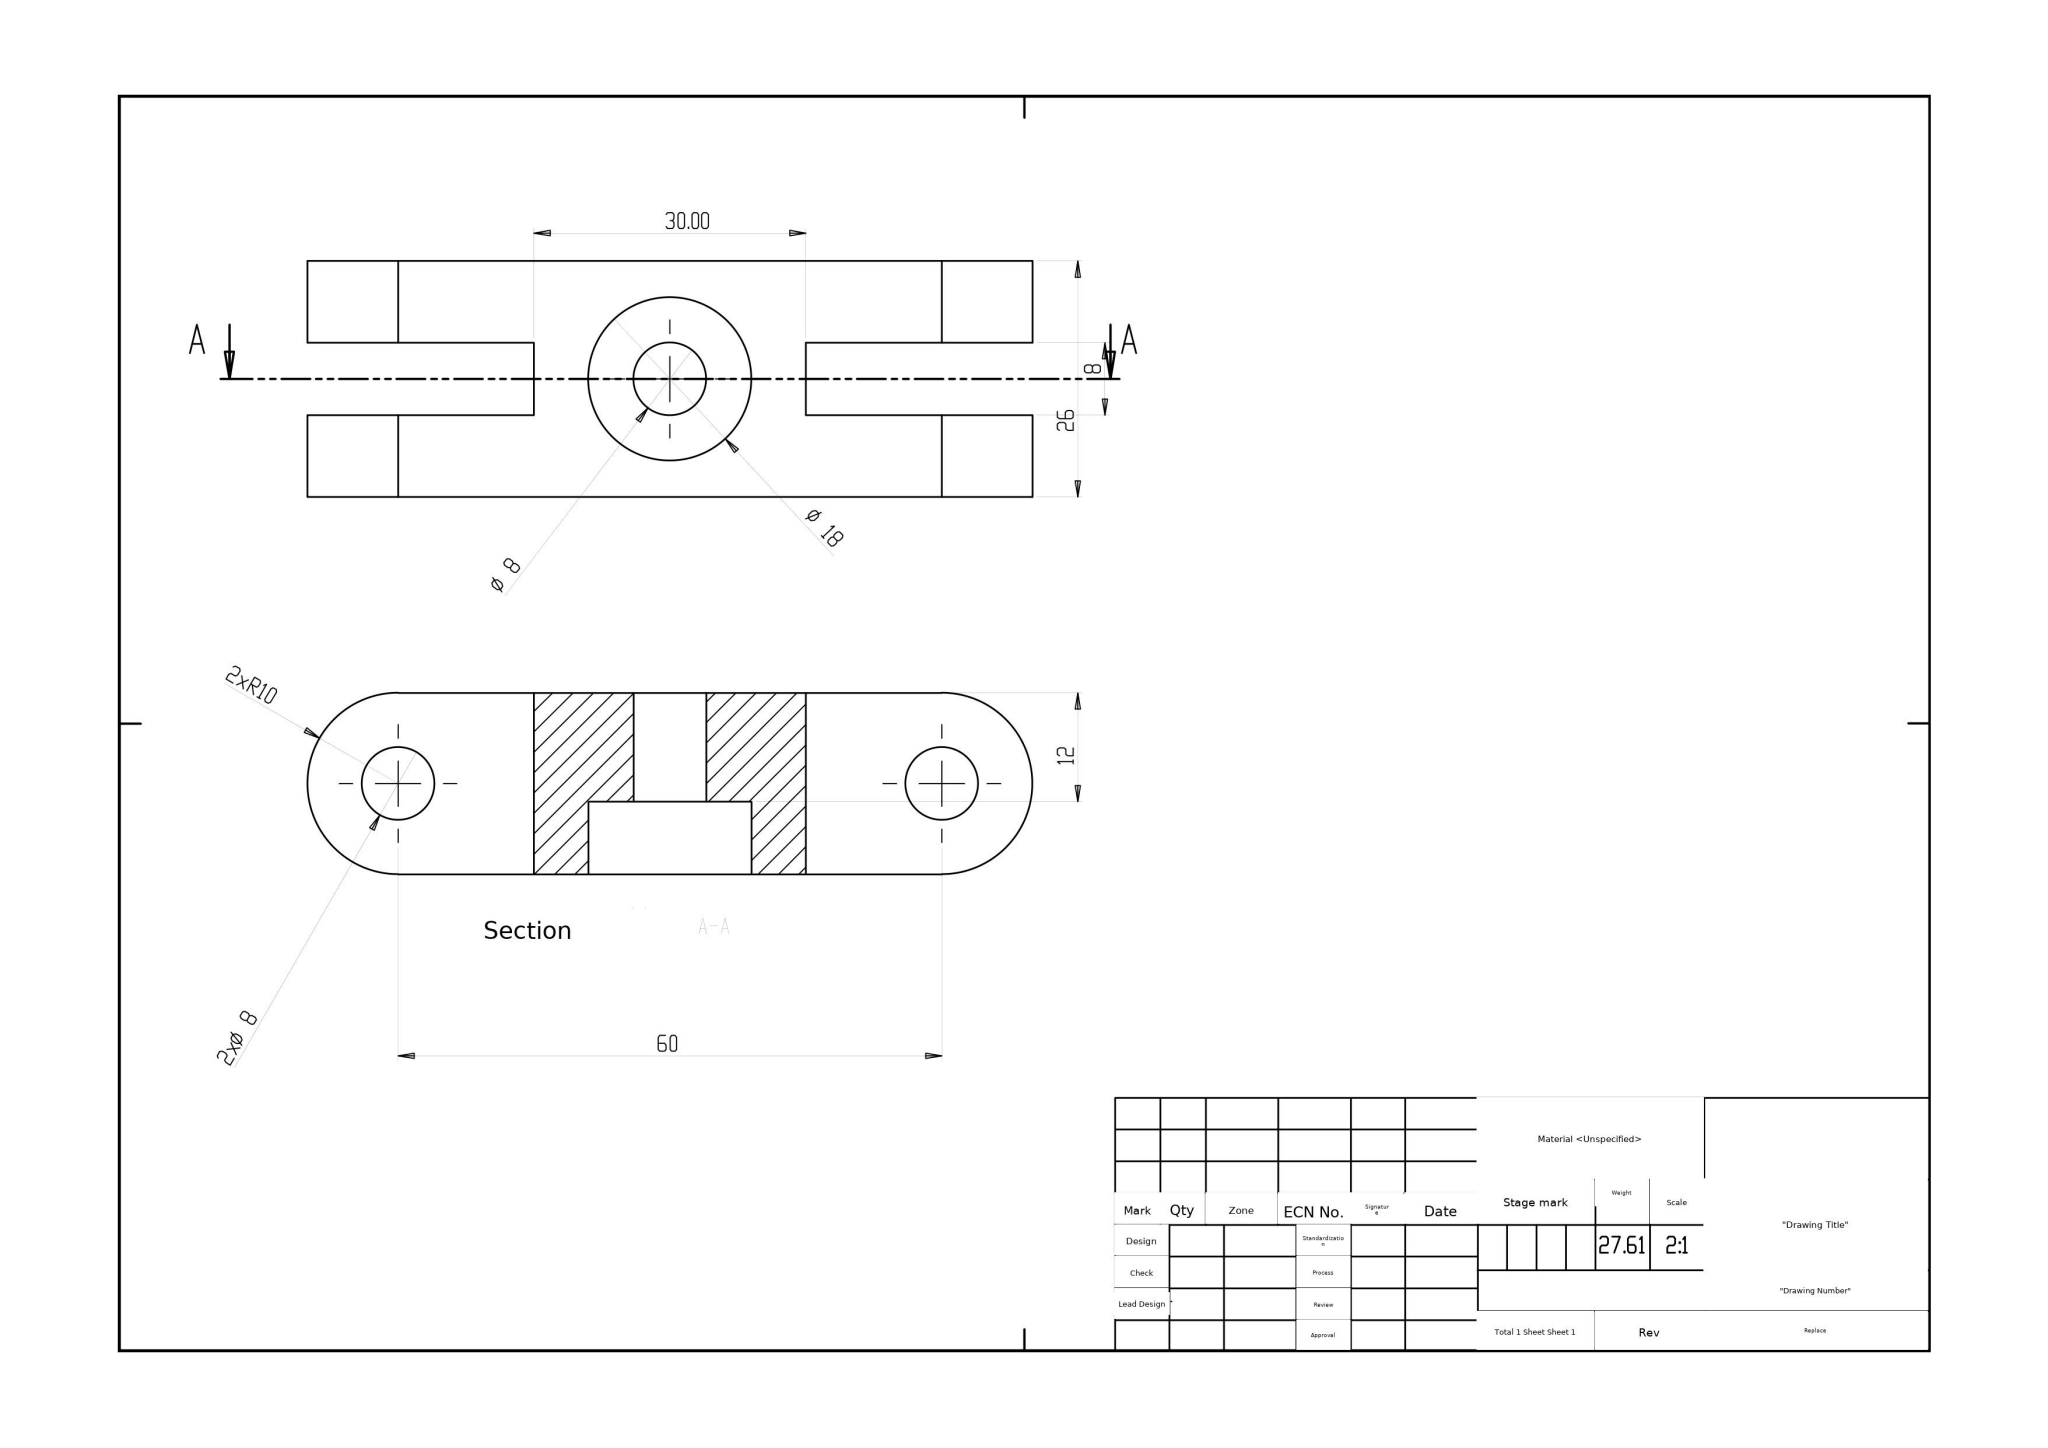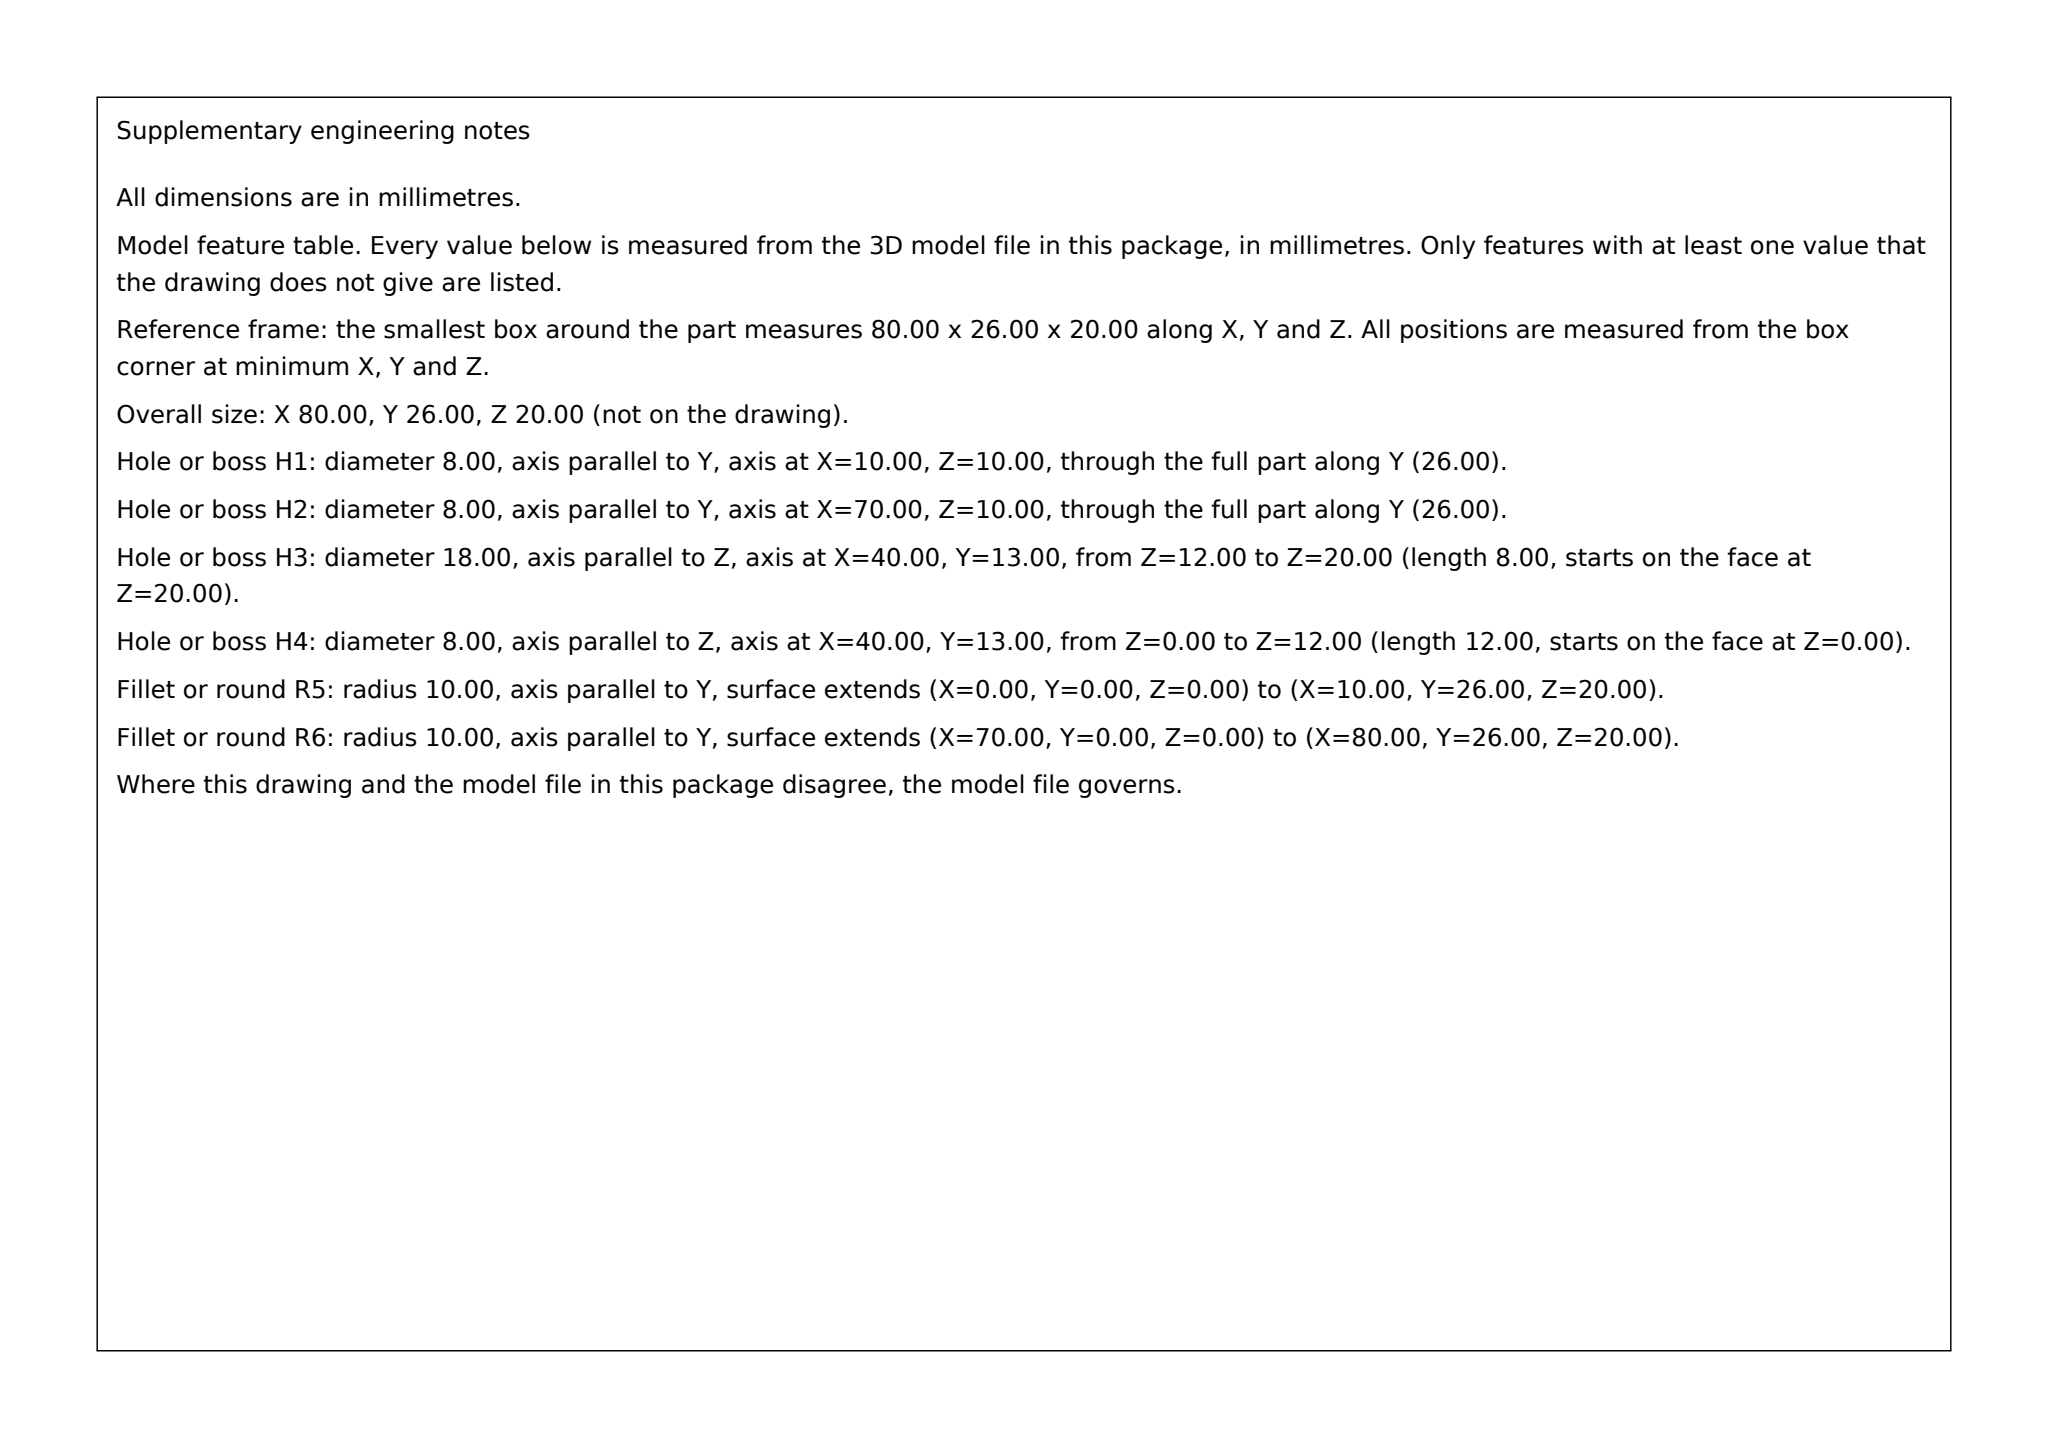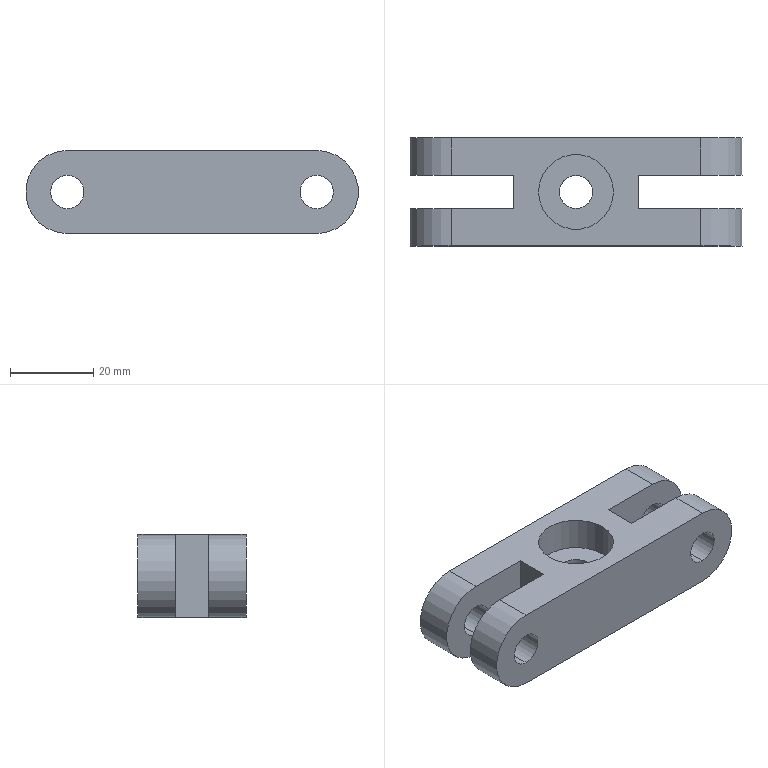Part | SolidWorks | mm | 1 solid | 27 faces | box 80 x 26 x 20 mm | volume 27606 mm3 | cylinder 16 | plane 11 | commonest cylinder face diameters 8 x10 20 x4 18 x2
build123d program:
from build123d import *

# Parameters (mm, degrees)
SKETCH1_R           = 4
BOSS_EXTRUDE1_DEPTH = 13
SKETCH2_W           = 25
SKETCH2_H           = 8
CUT_EXTRUDE1_DEPTH  = 47.573
HOLE1_D             = 8
HOLE1_CBORE_D       = 18
HOLE1_CBORE_DEPTH   = 8


with BuildPart() as part:
    # Sketch1 → Boss-Extrude1 (new, symmetric)
    with BuildSketch(Plane(origin=(0, 0, 0), x_dir=(1, 0, 0), z_dir=(0, 1, 0))):
        with BuildLine():
            Line((-30, 10), (30, 10))
            ThreePointArc((30, 10), (40, 0), (30, -10))
            Line((30, -10), (-30, -10))
            ThreePointArc((-30, -10), (-40, 0), (-30, 10))
        make_face()
        with Locations(Location((-30, 0, 0), (0, 0, 90))):
            Circle(SKETCH1_R, mode=Mode.SUBTRACT)
        with Locations(Location((30, 0, 0), (0, 0, 90))):
            Circle(SKETCH1_R, mode=Mode.SUBTRACT)
    extrude(amount=BOSS_EXTRUDE1_DEPTH, both=True)

    # Sketch2 → Cut-Extrude1 (cut, through all)
    with BuildSketch(Plane.XY.offset(10)):
        with Locations((27.5, 0)):
            Rectangle(SKETCH2_W, SKETCH2_H)
        with Locations((-27.5, 0)):
            Rectangle(SKETCH2_W, SKETCH2_H)
    extrude(amount=-CUT_EXTRUDE1_DEPTH, mode=Mode.SUBTRACT)

    # Hole1 (through all)
    with Locations(Plane.XY.offset(10)):
        with Locations((0, 0)):
            CounterBoreHole(HOLE1_D / 2, HOLE1_CBORE_D / 2, HOLE1_CBORE_DEPTH)


solid = part.part
STEP:
#1=CARTESIAN_POINT('',(-9.,0.,2.));
#2=VERTEX_POINT('',#1);
#3=CARTESIAN_POINT('',(9.,0.,2.));
#4=VERTEX_POINT('',#3);
#5=CARTESIAN_POINT('',(-0.,0.,2.));
#6=DIRECTION('',(0.,0.,1.));
#7=DIRECTION('',(1.,0.,0.));
#8=AXIS2_PLACEMENT_3D('',#5,#6,#7);
#9=CIRCLE('',#8,9.);
#10=EDGE_CURVE('',#2,#4,#9,.T.);
#11=ORIENTED_EDGE('',*,*,#10,.F.);
#12=CARTESIAN_POINT('',(-9.,0.,10.));
#13=VERTEX_POINT('',#12);
#14=CARTESIAN_POINT('',(-9.,0.,10.));
#15=DIRECTION('',(0.,0.,1.));
#16=VECTOR('',#15,1000.);
#17=LINE('',#14,#16);
#18=EDGE_CURVE('',#2,#13,#17,.T.);
#19=ORIENTED_EDGE('',*,*,#18,.T.);
#20=CARTESIAN_POINT('',(9.,0.,10.));
#21=VERTEX_POINT('',#20);
#22=CARTESIAN_POINT('',(-0.,0.,10.));
#23=DIRECTION('',(0.,0.,1.));
#24=DIRECTION('',(1.,0.,0.));
#25=AXIS2_PLACEMENT_3D('',#22,#23,#24);
#26=CIRCLE('',#25,9.);
#27=EDGE_CURVE('',#13,#21,#26,.T.);
#28=ORIENTED_EDGE('',*,*,#27,.T.);
#29=CARTESIAN_POINT('',(9.,0.,10.));
#30=DIRECTION('',(0.,0.,1.));
#31=VECTOR('',#30,1000.);
#32=LINE('',#29,#31);
#33=EDGE_CURVE('',#4,#21,#32,.T.);
#34=ORIENTED_EDGE('',*,*,#33,.F.);
#35=EDGE_LOOP('',(#11,#19,#28,#34));
#36=FACE_OUTER_BOUND('',#35,.T.);
#37=CARTESIAN_POINT('',(-0.,0.,10.));
#38=DIRECTION('',(0.,0.,1.));
#39=DIRECTION('',(1.,0.,0.));
#40=AXIS2_PLACEMENT_3D('',#37,#38,#39);
#41=CYLINDRICAL_SURFACE('',#40,9.);
#42=ADVANCED_FACE('',(#36),#41,.F.);
#43=CARTESIAN_POINT('',(-4.,0.,-10.));
#44=VERTEX_POINT('',#43);
#45=CARTESIAN_POINT('',(4.,0.,-10.));
#46=VERTEX_POINT('',#45);
#47=CARTESIAN_POINT('',(-0.,0.,-10.));
#48=DIRECTION('',(0.,0.,1.));
#49=DIRECTION('',(1.,0.,0.));
#50=AXIS2_PLACEMENT_3D('',#47,#48,#49);
#51=CIRCLE('',#50,4.);
#52=EDGE_CURVE('',#44,#46,#51,.T.);
#53=ORIENTED_EDGE('',*,*,#52,.F.);
#54=CARTESIAN_POINT('',(-4.,0.,2.));
#55=VERTEX_POINT('',#54);
#56=CARTESIAN_POINT('',(-4.,0.,10.));
#57=DIRECTION('',(0.,0.,1.));
#58=VECTOR('',#57,1000.);
#59=LINE('',#56,#58);
#60=EDGE_CURVE('',#44,#55,#59,.T.);
#61=ORIENTED_EDGE('',*,*,#60,.T.);
#62=CARTESIAN_POINT('',(4.,0.,2.));
#63=VERTEX_POINT('',#62);
#64=CARTESIAN_POINT('',(-0.,0.,2.));
#65=DIRECTION('',(0.,0.,1.));
#66=DIRECTION('',(1.,0.,0.));
#67=AXIS2_PLACEMENT_3D('',#64,#65,#66);
#68=CIRCLE('',#67,4.);
#69=EDGE_CURVE('',#55,#63,#68,.T.);
#70=ORIENTED_EDGE('',*,*,#69,.T.);
#71=CARTESIAN_POINT('',(4.,0.,10.));
#72=DIRECTION('',(0.,0.,1.));
#73=VECTOR('',#72,1000.);
#74=LINE('',#71,#73);
#75=EDGE_CURVE('',#46,#63,#74,.T.);
#76=ORIENTED_EDGE('',*,*,#75,.F.);
#77=EDGE_LOOP('',(#53,#61,#70,#76));
#78=FACE_OUTER_BOUND('',#77,.T.);
#79=CARTESIAN_POINT('',(-0.,0.,10.));
#80=DIRECTION('',(0.,0.,1.));
#81=DIRECTION('',(1.,0.,0.));
#82=AXIS2_PLACEMENT_3D('',#79,#80,#81);
#83=CYLINDRICAL_SURFACE('',#82,4.);
#84=ADVANCED_FACE('',(#78),#83,.F.);
#85=CARTESIAN_POINT('',(30.,13.,-4.));
#86=VERTEX_POINT('',#85);
#87=CARTESIAN_POINT('',(30.,13.,4.));
#88=VERTEX_POINT('',#87);
#89=CARTESIAN_POINT('',(30.,13.,0.));
#90=DIRECTION('',(0.,1.,0.));
#91=DIRECTION('',(0.,0.,1.));
#92=AXIS2_PLACEMENT_3D('',#89,#90,#91);
#93=CIRCLE('',#92,4.);
#94=EDGE_CURVE('',#86,#88,#93,.T.);
#95=ORIENTED_EDGE('',*,*,#94,.T.);
#96=CARTESIAN_POINT('',(30.,4.,4.));
#97=VERTEX_POINT('',#96);
#98=CARTESIAN_POINT('',(30.,13.,4.));
#99=DIRECTION('',(0.,-1.,0.));
#100=VECTOR('',#99,1000.);
#101=LINE('',#98,#100);
#102=EDGE_CURVE('',#88,#97,#101,.T.);
#103=ORIENTED_EDGE('',*,*,#102,.T.);
#104=CARTESIAN_POINT('',(30.,4.,-4.));
#105=VERTEX_POINT('',#104);
#106=CARTESIAN_POINT('',(30.,4.,0.));
#107=DIRECTION('',(0.,1.,0.));
#108=DIRECTION('',(0.,0.,1.));
#109=AXIS2_PLACEMENT_3D('',#106,#107,#108);
#110=CIRCLE('',#109,4.);
#111=EDGE_CURVE('',#105,#97,#110,.T.);
#112=ORIENTED_EDGE('',*,*,#111,.F.);
#113=CARTESIAN_POINT('',(30.,13.,-4.));
#114=DIRECTION('',(0.,-1.,0.));
#115=VECTOR('',#114,1000.);
#116=LINE('',#113,#115);
#117=EDGE_CURVE('',#86,#105,#116,.T.);
#118=ORIENTED_EDGE('',*,*,#117,.F.);
#119=EDGE_LOOP('',(#95,#103,#112,#118));
#120=FACE_OUTER_BOUND('',#119,.T.);
#121=CARTESIAN_POINT('',(30.,13.,0.));
#122=DIRECTION('',(0.,-1.,0.));
#123=DIRECTION('',(0.,0.,-1.));
#124=AXIS2_PLACEMENT_3D('',#121,#122,#123);
#125=CYLINDRICAL_SURFACE('',#124,4.);
#126=ADVANCED_FACE('',(#120),#125,.F.);
#127=CARTESIAN_POINT('',(-30.,13.,-4.));
#128=VERTEX_POINT('',#127);
#129=CARTESIAN_POINT('',(-30.,13.,4.));
#130=VERTEX_POINT('',#129);
#131=CARTESIAN_POINT('',(-30.,13.,0.));
#132=DIRECTION('',(0.,1.,0.));
#133=DIRECTION('',(0.,0.,1.));
#134=AXIS2_PLACEMENT_3D('',#131,#132,#133);
#135=CIRCLE('',#134,4.);
#136=EDGE_CURVE('',#128,#130,#135,.T.);
#137=ORIENTED_EDGE('',*,*,#136,.T.);
#138=CARTESIAN_POINT('',(-30.,4.,4.));
#139=VERTEX_POINT('',#138);
#140=CARTESIAN_POINT('',(-30.,13.,4.));
#141=DIRECTION('',(0.,-1.,0.));
#142=VECTOR('',#141,1000.);
#143=LINE('',#140,#142);
#144=EDGE_CURVE('',#130,#139,#143,.T.);
#145=ORIENTED_EDGE('',*,*,#144,.T.);
#146=CARTESIAN_POINT('',(-30.,4.,-4.));
#147=VERTEX_POINT('',#146);
#148=CARTESIAN_POINT('',(-30.,4.,0.));
#149=DIRECTION('',(-0.,1.,0.));
#150=DIRECTION('',(-1.,-0.,0.));
#151=AXIS2_PLACEMENT_3D('',#148,#149,#150);
#152=CIRCLE('',#151,4.);
#153=EDGE_CURVE('',#147,#139,#152,.T.);
#154=ORIENTED_EDGE('',*,*,#153,.F.);
#155=CARTESIAN_POINT('',(-30.,13.,-4.));
#156=DIRECTION('',(0.,-1.,0.));
#157=VECTOR('',#156,1000.);
#158=LINE('',#155,#157);
#159=EDGE_CURVE('',#128,#147,#158,.T.);
#160=ORIENTED_EDGE('',*,*,#159,.F.);
#161=EDGE_LOOP('',(#137,#145,#154,#160));
#162=FACE_OUTER_BOUND('',#161,.T.);
#163=CARTESIAN_POINT('',(-30.,13.,0.));
#164=DIRECTION('',(0.,-1.,0.));
#165=DIRECTION('',(0.,0.,-1.));
#166=AXIS2_PLACEMENT_3D('',#163,#164,#165);
#167=CYLINDRICAL_SURFACE('',#166,4.);
#168=ADVANCED_FACE('',(#162),#167,.F.);
#169=CARTESIAN_POINT('',(30.,-4.,4.));
#170=VERTEX_POINT('',#169);
#171=CARTESIAN_POINT('',(30.,-4.,-4.));
#172=VERTEX_POINT('',#171);
#173=CARTESIAN_POINT('',(30.,-4.,0.));
#174=DIRECTION('',(0.,-1.,0.));
#175=DIRECTION('',(0.,0.,-1.));
#176=AXIS2_PLACEMENT_3D('',#173,#174,#175);
#177=CIRCLE('',#176,4.);
#178=EDGE_CURVE('',#170,#172,#177,.T.);
#179=ORIENTED_EDGE('',*,*,#178,.F.);
#180=CARTESIAN_POINT('',(30.,-13.,4.));
#181=VERTEX_POINT('',#180);
#182=CARTESIAN_POINT('',(30.,13.,4.));
#183=DIRECTION('',(0.,-1.,0.));
#184=VECTOR('',#183,1000.);
#185=LINE('',#182,#184);
#186=EDGE_CURVE('',#170,#181,#185,.T.);
#187=ORIENTED_EDGE('',*,*,#186,.T.);
#188=CARTESIAN_POINT('',(30.,-13.,-4.));
#189=VERTEX_POINT('',#188);
#190=CARTESIAN_POINT('',(30.,-13.,0.));
#191=DIRECTION('',(0.,1.,0.));
#192=DIRECTION('',(0.,0.,1.));
#193=AXIS2_PLACEMENT_3D('',#190,#191,#192);
#194=CIRCLE('',#193,4.);
#195=EDGE_CURVE('',#189,#181,#194,.T.);
#196=ORIENTED_EDGE('',*,*,#195,.F.);
#197=CARTESIAN_POINT('',(30.,13.,-4.));
#198=DIRECTION('',(0.,-1.,0.));
#199=VECTOR('',#198,1000.);
#200=LINE('',#197,#199);
#201=EDGE_CURVE('',#172,#189,#200,.T.);
#202=ORIENTED_EDGE('',*,*,#201,.F.);
#203=EDGE_LOOP('',(#179,#187,#196,#202));
#204=FACE_OUTER_BOUND('',#203,.T.);
#205=CARTESIAN_POINT('',(30.,13.,0.));
#206=DIRECTION('',(0.,-1.,0.));
#207=DIRECTION('',(0.,0.,-1.));
#208=AXIS2_PLACEMENT_3D('',#205,#206,#207);
#209=CYLINDRICAL_SURFACE('',#208,4.);
#210=ADVANCED_FACE('',(#204),#209,.F.);
#211=CARTESIAN_POINT('',(-30.,-4.,4.));
#212=VERTEX_POINT('',#211);
#213=CARTESIAN_POINT('',(-30.,-4.,-4.));
#214=VERTEX_POINT('',#213);
#215=CARTESIAN_POINT('',(-30.,-4.,0.));
#216=DIRECTION('',(0.,-1.,0.));
#217=DIRECTION('',(1.,0.,0.));
#218=AXIS2_PLACEMENT_3D('',#215,#216,#217);
#219=CIRCLE('',#218,4.);
#220=EDGE_CURVE('',#212,#214,#219,.T.);
#221=ORIENTED_EDGE('',*,*,#220,.F.);
#222=CARTESIAN_POINT('',(-30.,-13.,4.));
#223=VERTEX_POINT('',#222);
#224=CARTESIAN_POINT('',(-30.,13.,4.));
#225=DIRECTION('',(0.,-1.,0.));
#226=VECTOR('',#225,1000.);
#227=LINE('',#224,#226);
#228=EDGE_CURVE('',#212,#223,#227,.T.);
#229=ORIENTED_EDGE('',*,*,#228,.T.);
#230=CARTESIAN_POINT('',(-30.,-13.,-4.));
#231=VERTEX_POINT('',#230);
#232=CARTESIAN_POINT('',(-30.,-13.,0.));
#233=DIRECTION('',(0.,1.,0.));
#234=DIRECTION('',(0.,0.,1.));
#235=AXIS2_PLACEMENT_3D('',#232,#233,#234);
#236=CIRCLE('',#235,4.);
#237=EDGE_CURVE('',#231,#223,#236,.T.);
#238=ORIENTED_EDGE('',*,*,#237,.F.);
#239=CARTESIAN_POINT('',(-30.,13.,-4.));
#240=DIRECTION('',(0.,-1.,0.));
#241=VECTOR('',#240,1000.);
#242=LINE('',#239,#241);
#243=EDGE_CURVE('',#214,#231,#242,.T.);
#244=ORIENTED_EDGE('',*,*,#243,.F.);
#245=EDGE_LOOP('',(#221,#229,#238,#244));
#246=FACE_OUTER_BOUND('',#245,.T.);
#247=CARTESIAN_POINT('',(-30.,13.,0.));
#248=DIRECTION('',(0.,-1.,0.));
#249=DIRECTION('',(0.,0.,-1.));
#250=AXIS2_PLACEMENT_3D('',#247,#248,#249);
#251=CYLINDRICAL_SURFACE('',#250,4.);
#252=ADVANCED_FACE('',(#246),#251,.F.);
#253=CARTESIAN_POINT('',(-30.,-4.,10.));
#254=VERTEX_POINT('',#253);
#255=CARTESIAN_POINT('',(-30.,-13.,10.));
#256=VERTEX_POINT('',#255);
#257=CARTESIAN_POINT('',(-30.,13.,10.));
#258=DIRECTION('',(0.,-1.,0.));
#259=VECTOR('',#258,1000.);
#260=LINE('',#257,#259);
#261=EDGE_CURVE('',#254,#256,#260,.T.);
#262=ORIENTED_EDGE('',*,*,#261,.F.);
#263=CARTESIAN_POINT('',(-30.,-4.,-10.));
#264=VERTEX_POINT('',#263);
#265=CARTESIAN_POINT('',(-30.,-4.,0.));
#266=DIRECTION('',(0.,-1.,0.));
#267=DIRECTION('',(1.,0.,0.));
#268=AXIS2_PLACEMENT_3D('',#265,#266,#267);
#269=CIRCLE('',#268,10.);
#270=EDGE_CURVE('',#254,#264,#269,.T.);
#271=ORIENTED_EDGE('',*,*,#270,.T.);
#272=CARTESIAN_POINT('',(-30.,-13.,-10.));
#273=VERTEX_POINT('',#272);
#274=CARTESIAN_POINT('',(-30.,13.,-10.));
#275=DIRECTION('',(0.,-1.,0.));
#276=VECTOR('',#275,1000.);
#277=LINE('',#274,#276);
#278=EDGE_CURVE('',#264,#273,#277,.T.);
#279=ORIENTED_EDGE('',*,*,#278,.T.);
#280=CARTESIAN_POINT('',(-30.,-13.,0.));
#281=DIRECTION('',(0.,1.,0.));
#282=DIRECTION('',(0.,0.,1.));
#283=AXIS2_PLACEMENT_3D('',#280,#281,#282);
#284=CIRCLE('',#283,10.);
#285=EDGE_CURVE('',#273,#256,#284,.T.);
#286=ORIENTED_EDGE('',*,*,#285,.T.);
#287=EDGE_LOOP('',(#262,#271,#279,#286));
#288=FACE_OUTER_BOUND('',#287,.T.);
#289=CARTESIAN_POINT('',(-30.,13.,0.));
#290=DIRECTION('',(0.,-1.,0.));
#291=DIRECTION('',(0.,0.,-1.));
#292=AXIS2_PLACEMENT_3D('',#289,#290,#291);
#293=CYLINDRICAL_SURFACE('',#292,10.);
#294=ADVANCED_FACE('',(#288),#293,.T.);
#295=CARTESIAN_POINT('',(30.,-4.,-10.));
#296=VERTEX_POINT('',#295);
#297=CARTESIAN_POINT('',(30.,-13.,-10.));
#298=VERTEX_POINT('',#297);
#299=CARTESIAN_POINT('',(30.,13.,-10.));
#300=DIRECTION('',(0.,-1.,0.));
#301=VECTOR('',#300,1000.);
#302=LINE('',#299,#301);
#303=EDGE_CURVE('',#296,#298,#302,.T.);
#304=ORIENTED_EDGE('',*,*,#303,.F.);
#305=CARTESIAN_POINT('',(30.,-4.,10.));
#306=VERTEX_POINT('',#305);
#307=CARTESIAN_POINT('',(30.,-4.,0.));
#308=DIRECTION('',(0.,-1.,0.));
#309=DIRECTION('',(0.,0.,-1.));
#310=AXIS2_PLACEMENT_3D('',#307,#308,#309);
#311=CIRCLE('',#310,10.);
#312=EDGE_CURVE('',#296,#306,#311,.T.);
#313=ORIENTED_EDGE('',*,*,#312,.T.);
#314=CARTESIAN_POINT('',(30.,-13.,10.));
#315=VERTEX_POINT('',#314);
#316=CARTESIAN_POINT('',(30.,13.,10.));
#317=DIRECTION('',(0.,-1.,0.));
#318=VECTOR('',#317,1000.);
#319=LINE('',#316,#318);
#320=EDGE_CURVE('',#306,#315,#319,.T.);
#321=ORIENTED_EDGE('',*,*,#320,.T.);
#322=CARTESIAN_POINT('',(30.,-13.,0.));
#323=DIRECTION('',(0.,1.,0.));
#324=DIRECTION('',(0.,0.,1.));
#325=AXIS2_PLACEMENT_3D('',#322,#323,#324);
#326=CIRCLE('',#325,10.);
#327=EDGE_CURVE('',#315,#298,#326,.T.);
#328=ORIENTED_EDGE('',*,*,#327,.T.);
#329=EDGE_LOOP('',(#304,#313,#321,#328));
#330=FACE_OUTER_BOUND('',#329,.T.);
#331=CARTESIAN_POINT('',(30.,13.,0.));
#332=DIRECTION('',(0.,-1.,0.));
#333=DIRECTION('',(0.,0.,-1.));
#334=AXIS2_PLACEMENT_3D('',#331,#332,#333);
#335=CYLINDRICAL_SURFACE('',#334,10.);
#336=ADVANCED_FACE('',(#330),#335,.T.);
#337=ORIENTED_EDGE('',*,*,#228,.F.);
#338=CARTESIAN_POINT('',(-30.,-4.,0.));
#339=DIRECTION('',(0.,-1.,0.));
#340=DIRECTION('',(1.,0.,0.));
#341=AXIS2_PLACEMENT_3D('',#338,#339,#340);
#342=CIRCLE('',#341,4.);
#343=EDGE_CURVE('',#214,#212,#342,.T.);
#344=ORIENTED_EDGE('',*,*,#343,.F.);
#345=ORIENTED_EDGE('',*,*,#243,.T.);
#346=CARTESIAN_POINT('',(-30.,-13.,0.));
#347=DIRECTION('',(0.,1.,0.));
#348=DIRECTION('',(0.,0.,1.));
#349=AXIS2_PLACEMENT_3D('',#346,#347,#348);
#350=CIRCLE('',#349,4.);
#351=EDGE_CURVE('',#223,#231,#350,.T.);
#352=ORIENTED_EDGE('',*,*,#351,.F.);
#353=EDGE_LOOP('',(#337,#344,#345,#352));
#354=FACE_OUTER_BOUND('',#353,.T.);
#355=CARTESIAN_POINT('',(-30.,13.,0.));
#356=DIRECTION('',(0.,-1.,0.));
#357=DIRECTION('',(0.,0.,-1.));
#358=AXIS2_PLACEMENT_3D('',#355,#356,#357);
#359=CYLINDRICAL_SURFACE('',#358,4.);
#360=ADVANCED_FACE('',(#354),#359,.F.);
#361=ORIENTED_EDGE('',*,*,#186,.F.);
#362=CARTESIAN_POINT('',(30.,-4.,0.));
#363=DIRECTION('',(0.,-1.,0.));
#364=DIRECTION('',(0.,0.,-1.));
#365=AXIS2_PLACEMENT_3D('',#362,#363,#364);
#366=CIRCLE('',#365,4.);
#367=EDGE_CURVE('',#172,#170,#366,.T.);
#368=ORIENTED_EDGE('',*,*,#367,.F.);
#369=ORIENTED_EDGE('',*,*,#201,.T.);
#370=CARTESIAN_POINT('',(30.,-13.,0.));
#371=DIRECTION('',(0.,1.,0.));
#372=DIRECTION('',(0.,0.,1.));
#373=AXIS2_PLACEMENT_3D('',#370,#371,#372);
#374=CIRCLE('',#373,4.);
#375=EDGE_CURVE('',#181,#189,#374,.T.);
#376=ORIENTED_EDGE('',*,*,#375,.F.);
#377=EDGE_LOOP('',(#361,#368,#369,#376));
#378=FACE_OUTER_BOUND('',#377,.T.);
#379=CARTESIAN_POINT('',(30.,13.,0.));
#380=DIRECTION('',(0.,-1.,0.));
#381=DIRECTION('',(0.,0.,-1.));
#382=AXIS2_PLACEMENT_3D('',#379,#380,#381);
#383=CYLINDRICAL_SURFACE('',#382,4.);
#384=ADVANCED_FACE('',(#378),#383,.F.);
#385=ORIENTED_EDGE('',*,*,#136,.F.);
#386=CARTESIAN_POINT('',(-30.,13.,0.));
#387=DIRECTION('',(0.,1.,0.));
#388=DIRECTION('',(0.,0.,1.));
#389=AXIS2_PLACEMENT_3D('',#386,#387,#388);
#390=CIRCLE('',#389,4.);
#391=EDGE_CURVE('',#130,#128,#390,.T.);
#392=ORIENTED_EDGE('',*,*,#391,.F.);
#393=EDGE_LOOP('',(#385,#392));
#394=FACE_BOUND('',#393,.T.);
#395=CARTESIAN_POINT('',(-30.,13.,-10.));
#396=VERTEX_POINT('',#395);
#397=CARTESIAN_POINT('',(-30.,13.,10.));
#398=VERTEX_POINT('',#397);
#399=CARTESIAN_POINT('',(-30.,13.,0.));
#400=DIRECTION('',(0.,1.,0.));
#401=DIRECTION('',(0.,0.,1.));
#402=AXIS2_PLACEMENT_3D('',#399,#400,#401);
#403=CIRCLE('',#402,10.);
#404=EDGE_CURVE('',#396,#398,#403,.T.);
#405=ORIENTED_EDGE('',*,*,#404,.T.);
#406=CARTESIAN_POINT('',(30.,13.,10.));
#407=VERTEX_POINT('',#406);
#408=CARTESIAN_POINT('',(-30.,13.,10.));
#409=DIRECTION('',(1.,0.,-0.));
#410=VECTOR('',#409,1000.);
#411=LINE('',#408,#410);
#412=EDGE_CURVE('',#398,#407,#411,.T.);
#413=ORIENTED_EDGE('',*,*,#412,.T.);
#414=CARTESIAN_POINT('',(30.,13.,-10.));
#415=VERTEX_POINT('',#414);
#416=CARTESIAN_POINT('',(30.,13.,0.));
#417=DIRECTION('',(0.,1.,0.));
#418=DIRECTION('',(0.,0.,1.));
#419=AXIS2_PLACEMENT_3D('',#416,#417,#418);
#420=CIRCLE('',#419,10.);
#421=EDGE_CURVE('',#407,#415,#420,.T.);
#422=ORIENTED_EDGE('',*,*,#421,.T.);
#423=CARTESIAN_POINT('',(-30.,13.,-10.));
#424=DIRECTION('',(-1.,0.,0.));
#425=VECTOR('',#424,1000.);
#426=LINE('',#423,#425);
#427=EDGE_CURVE('',#415,#396,#426,.T.);
#428=ORIENTED_EDGE('',*,*,#427,.T.);
#429=EDGE_LOOP('',(#405,#413,#422,#428));
#430=FACE_OUTER_BOUND('',#429,.T.);
#431=ORIENTED_EDGE('',*,*,#94,.F.);
#432=CARTESIAN_POINT('',(30.,13.,0.));
#433=DIRECTION('',(0.,1.,0.));
#434=DIRECTION('',(0.,0.,1.));
#435=AXIS2_PLACEMENT_3D('',#432,#433,#434);
#436=CIRCLE('',#435,4.);
#437=EDGE_CURVE('',#88,#86,#436,.T.);
#438=ORIENTED_EDGE('',*,*,#437,.F.);
#439=EDGE_LOOP('',(#431,#438));
#440=FACE_BOUND('',#439,.T.);
#441=CARTESIAN_POINT('',(-30.,13.,0.));
#442=DIRECTION('',(0.,1.,0.));
#443=DIRECTION('',(0.,0.,1.));
#444=AXIS2_PLACEMENT_3D('',#441,#442,#443);
#445=PLANE('',#444);
#446=ADVANCED_FACE('',(#394,#430,#440),#445,.T.);
#447=ORIENTED_EDGE('',*,*,#285,.F.);
#448=CARTESIAN_POINT('',(-30.,-13.,-10.));
#449=DIRECTION('',(-1.,0.,0.));
#450=VECTOR('',#449,1000.);
#451=LINE('',#448,#450);
#452=EDGE_CURVE('',#298,#273,#451,.T.);
#453=ORIENTED_EDGE('',*,*,#452,.F.);
#454=ORIENTED_EDGE('',*,*,#327,.F.);
#455=CARTESIAN_POINT('',(-30.,-13.,10.));
#456=DIRECTION('',(1.,0.,-0.));
#457=VECTOR('',#456,1000.);
#458=LINE('',#455,#457);
#459=EDGE_CURVE('',#256,#315,#458,.T.);
#460=ORIENTED_EDGE('',*,*,#459,.F.);
#461=EDGE_LOOP('',(#447,#453,#454,#460));
#462=FACE_OUTER_BOUND('',#461,.T.);
#463=ORIENTED_EDGE('',*,*,#237,.T.);
#464=ORIENTED_EDGE('',*,*,#351,.T.);
#465=EDGE_LOOP('',(#463,#464));
#466=FACE_BOUND('',#465,.T.);
#467=ORIENTED_EDGE('',*,*,#195,.T.);
#468=ORIENTED_EDGE('',*,*,#375,.T.);
#469=EDGE_LOOP('',(#467,#468));
#470=FACE_BOUND('',#469,.T.);
#471=CARTESIAN_POINT('',(-30.,-13.,0.));
#472=DIRECTION('',(0.,1.,0.));
#473=DIRECTION('',(0.,0.,1.));
#474=AXIS2_PLACEMENT_3D('',#471,#472,#473);
#475=PLANE('',#474);
#476=ADVANCED_FACE('',(#462,#466,#470),#475,.F.);
#477=CARTESIAN_POINT('',(-30.,4.,-10.));
#478=VERTEX_POINT('',#477);
#479=CARTESIAN_POINT('',(-30.,4.,10.));
#480=VERTEX_POINT('',#479);
#481=CARTESIAN_POINT('',(-30.,4.,0.));
#482=DIRECTION('',(-0.,1.,0.));
#483=DIRECTION('',(-1.,-0.,0.));
#484=AXIS2_PLACEMENT_3D('',#481,#482,#483);
#485=CIRCLE('',#484,10.);
#486=EDGE_CURVE('',#478,#480,#485,.T.);
#487=ORIENTED_EDGE('',*,*,#486,.T.);
#488=CARTESIAN_POINT('',(-30.,13.,10.));
#489=DIRECTION('',(0.,-1.,0.));
#490=VECTOR('',#489,1000.);
#491=LINE('',#488,#490);
#492=EDGE_CURVE('',#398,#480,#491,.T.);
#493=ORIENTED_EDGE('',*,*,#492,.F.);
#494=ORIENTED_EDGE('',*,*,#404,.F.);
#495=CARTESIAN_POINT('',(-30.,13.,-10.));
#496=DIRECTION('',(0.,-1.,0.));
#497=VECTOR('',#496,1000.);
#498=LINE('',#495,#497);
#499=EDGE_CURVE('',#396,#478,#498,.T.);
#500=ORIENTED_EDGE('',*,*,#499,.T.);
#501=EDGE_LOOP('',(#487,#493,#494,#500));
#502=FACE_OUTER_BOUND('',#501,.T.);
#503=CARTESIAN_POINT('',(-30.,13.,0.));
#504=DIRECTION('',(0.,-1.,0.));
#505=DIRECTION('',(0.,0.,-1.));
#506=AXIS2_PLACEMENT_3D('',#503,#504,#505);
#507=CYLINDRICAL_SURFACE('',#506,10.);
#508=ADVANCED_FACE('',(#502),#507,.T.);
#509=CARTESIAN_POINT('',(-0.,0.,10.));
#510=DIRECTION('',(0.,0.,1.));
#511=DIRECTION('',(1.,0.,0.));
#512=AXIS2_PLACEMENT_3D('',#509,#510,#511);
#513=CIRCLE('',#512,9.);
#514=EDGE_CURVE('',#21,#13,#513,.T.);
#515=ORIENTED_EDGE('',*,*,#514,.F.);
#516=ORIENTED_EDGE('',*,*,#27,.F.);
#517=EDGE_LOOP('',(#515,#516));
#518=FACE_BOUND('',#517,.T.);
#519=ORIENTED_EDGE('',*,*,#320,.F.);
#520=CARTESIAN_POINT('',(15.,-4.,10.));
#521=VERTEX_POINT('',#520);
#522=CARTESIAN_POINT('',(15.,-4.,10.));
#523=DIRECTION('',(1.,0.,0.));
#524=VECTOR('',#523,1000.);
#525=LINE('',#522,#524);
#526=EDGE_CURVE('',#521,#306,#525,.T.);
#527=ORIENTED_EDGE('',*,*,#526,.F.);
#528=CARTESIAN_POINT('',(15.,4.,10.));
#529=VERTEX_POINT('',#528);
#530=CARTESIAN_POINT('',(15.,4.,10.));
#531=DIRECTION('',(0.,-1.,0.));
#532=VECTOR('',#531,1000.);
#533=LINE('',#530,#532);
#534=EDGE_CURVE('',#529,#521,#533,.T.);
#535=ORIENTED_EDGE('',*,*,#534,.F.);
#536=CARTESIAN_POINT('',(30.,4.,10.));
#537=VERTEX_POINT('',#536);
#538=CARTESIAN_POINT('',(15.,4.,10.));
#539=DIRECTION('',(-1.,0.,0.));
#540=VECTOR('',#539,1000.);
#541=LINE('',#538,#540);
#542=EDGE_CURVE('',#537,#529,#541,.T.);
#543=ORIENTED_EDGE('',*,*,#542,.F.);
#544=CARTESIAN_POINT('',(30.,13.,10.));
#545=DIRECTION('',(0.,-1.,0.));
#546=VECTOR('',#545,1000.);
#547=LINE('',#544,#546);
#548=EDGE_CURVE('',#407,#537,#547,.T.);
#549=ORIENTED_EDGE('',*,*,#548,.F.);
#550=ORIENTED_EDGE('',*,*,#412,.F.);
#551=ORIENTED_EDGE('',*,*,#492,.T.);
#552=CARTESIAN_POINT('',(-15.,4.,10.));
#553=VERTEX_POINT('',#552);
#554=CARTESIAN_POINT('',(-15.,4.,10.));
#555=DIRECTION('',(-1.,-0.,0.));
#556=VECTOR('',#555,1000.);
#557=LINE('',#554,#556);
#558=EDGE_CURVE('',#553,#480,#557,.T.);
#559=ORIENTED_EDGE('',*,*,#558,.F.);
#560=CARTESIAN_POINT('',(-15.,-4.,10.));
#561=VERTEX_POINT('',#560);
#562=CARTESIAN_POINT('',(-15.,4.,10.));
#563=DIRECTION('',(-0.,1.,0.));
#564=VECTOR('',#563,1000.);
#565=LINE('',#562,#564);
#566=EDGE_CURVE('',#561,#553,#565,.T.);
#567=ORIENTED_EDGE('',*,*,#566,.F.);
#568=CARTESIAN_POINT('',(-15.,-4.,10.));
#569=DIRECTION('',(1.,0.,0.));
#570=VECTOR('',#569,1000.);
#571=LINE('',#568,#570);
#572=EDGE_CURVE('',#254,#561,#571,.T.);
#573=ORIENTED_EDGE('',*,*,#572,.F.);
#574=ORIENTED_EDGE('',*,*,#261,.T.);
#575=ORIENTED_EDGE('',*,*,#459,.T.);
#576=EDGE_LOOP('',(#519,#527,#535,#543,#549,#550,#551,#559,#567,#573,#574,#575));
#577=FACE_OUTER_BOUND('',#576,.T.);
#578=CARTESIAN_POINT('',(-30.,13.,10.));
#579=DIRECTION('',(-0.,0.,-1.));
#580=DIRECTION('',(-1.,0.,0.));
#581=AXIS2_PLACEMENT_3D('',#578,#579,#580);
#582=PLANE('',#581);
#583=ADVANCED_FACE('',(#518,#577),#582,.F.);
#584=ORIENTED_EDGE('',*,*,#548,.T.);
#585=CARTESIAN_POINT('',(30.,4.,-10.));
#586=VERTEX_POINT('',#585);
#587=CARTESIAN_POINT('',(30.,4.,0.));
#588=DIRECTION('',(0.,1.,0.));
#589=DIRECTION('',(0.,0.,1.));
#590=AXIS2_PLACEMENT_3D('',#587,#588,#589);
#591=CIRCLE('',#590,10.);
#592=EDGE_CURVE('',#537,#586,#591,.T.);
#593=ORIENTED_EDGE('',*,*,#592,.T.);
#594=CARTESIAN_POINT('',(30.,13.,-10.));
#595=DIRECTION('',(0.,-1.,0.));
#596=VECTOR('',#595,1000.);
#597=LINE('',#594,#596);
#598=EDGE_CURVE('',#415,#586,#597,.T.);
#599=ORIENTED_EDGE('',*,*,#598,.F.);
#600=ORIENTED_EDGE('',*,*,#421,.F.);
#601=EDGE_LOOP('',(#584,#593,#599,#600));
#602=FACE_OUTER_BOUND('',#601,.T.);
#603=CARTESIAN_POINT('',(30.,13.,0.));
#604=DIRECTION('',(0.,-1.,0.));
#605=DIRECTION('',(0.,0.,-1.));
#606=AXIS2_PLACEMENT_3D('',#603,#604,#605);
#607=CYLINDRICAL_SURFACE('',#606,10.);
#608=ADVANCED_FACE('',(#602),#607,.T.);
#609=CARTESIAN_POINT('',(-0.,0.,-10.));
#610=DIRECTION('',(0.,0.,1.));
#611=DIRECTION('',(1.,0.,0.));
#612=AXIS2_PLACEMENT_3D('',#609,#610,#611);
#613=CIRCLE('',#612,4.);
#614=EDGE_CURVE('',#46,#44,#613,.T.);
#615=ORIENTED_EDGE('',*,*,#614,.T.);
#616=ORIENTED_EDGE('',*,*,#52,.T.);
#617=EDGE_LOOP('',(#615,#616));
#618=FACE_BOUND('',#617,.T.);
#619=CARTESIAN_POINT('',(15.,4.,-10.));
#620=VERTEX_POINT('',#619);
#621=CARTESIAN_POINT('',(15.,-4.,-10.));
#622=VERTEX_POINT('',#621);
#623=CARTESIAN_POINT('',(15.,4.,-10.));
#624=DIRECTION('',(0.,-1.,0.));
#625=VECTOR('',#624,1000.);
#626=LINE('',#623,#625);
#627=EDGE_CURVE('',#620,#622,#626,.T.);
#628=ORIENTED_EDGE('',*,*,#627,.T.);
#629=CARTESIAN_POINT('',(15.,-4.,-10.));
#630=DIRECTION('',(1.,0.,0.));
#631=VECTOR('',#630,1000.);
#632=LINE('',#629,#631);
#633=EDGE_CURVE('',#622,#296,#632,.T.);
#634=ORIENTED_EDGE('',*,*,#633,.T.);
#635=ORIENTED_EDGE('',*,*,#303,.T.);
#636=ORIENTED_EDGE('',*,*,#452,.T.);
#637=ORIENTED_EDGE('',*,*,#278,.F.);
#638=CARTESIAN_POINT('',(-15.,-4.,-10.));
#639=VERTEX_POINT('',#638);
#640=CARTESIAN_POINT('',(-15.,-4.,-10.));
#641=DIRECTION('',(1.,0.,0.));
#642=VECTOR('',#641,1000.);
#643=LINE('',#640,#642);
#644=EDGE_CURVE('',#264,#639,#643,.T.);
#645=ORIENTED_EDGE('',*,*,#644,.T.);
#646=CARTESIAN_POINT('',(-15.,4.,-10.));
#647=VERTEX_POINT('',#646);
#648=CARTESIAN_POINT('',(-15.,4.,-10.));
#649=DIRECTION('',(-0.,1.,0.));
#650=VECTOR('',#649,1000.);
#651=LINE('',#648,#650);
#652=EDGE_CURVE('',#639,#647,#651,.T.);
#653=ORIENTED_EDGE('',*,*,#652,.T.);
#654=CARTESIAN_POINT('',(-15.,4.,-10.));
#655=DIRECTION('',(-1.,-0.,0.));
#656=VECTOR('',#655,1000.);
#657=LINE('',#654,#656);
#658=EDGE_CURVE('',#647,#478,#657,.T.);
#659=ORIENTED_EDGE('',*,*,#658,.T.);
#660=ORIENTED_EDGE('',*,*,#499,.F.);
#661=ORIENTED_EDGE('',*,*,#427,.F.);
#662=ORIENTED_EDGE('',*,*,#598,.T.);
#663=CARTESIAN_POINT('',(15.,4.,-10.));
#664=DIRECTION('',(-1.,0.,0.));
#665=VECTOR('',#664,1000.);
#666=LINE('',#663,#665);
#667=EDGE_CURVE('',#586,#620,#666,.T.);
#668=ORIENTED_EDGE('',*,*,#667,.T.);
#669=EDGE_LOOP('',(#628,#634,#635,#636,#637,#645,#653,#659,#660,#661,#662,#668));
#670=FACE_OUTER_BOUND('',#669,.T.);
#671=CARTESIAN_POINT('',(-30.,13.,-10.));
#672=DIRECTION('',(0.,0.,1.));
#673=DIRECTION('',(1.,0.,-0.));
#674=AXIS2_PLACEMENT_3D('',#671,#672,#673);
#675=PLANE('',#674);
#676=ADVANCED_FACE('',(#618,#670),#675,.F.);
#677=ORIENTED_EDGE('',*,*,#144,.F.);
#678=ORIENTED_EDGE('',*,*,#391,.T.);
#679=ORIENTED_EDGE('',*,*,#159,.T.);
#680=CARTESIAN_POINT('',(-30.,4.,0.));
#681=DIRECTION('',(-0.,1.,0.));
#682=DIRECTION('',(-1.,-0.,0.));
#683=AXIS2_PLACEMENT_3D('',#680,#681,#682);
#684=CIRCLE('',#683,4.);
#685=EDGE_CURVE('',#139,#147,#684,.T.);
#686=ORIENTED_EDGE('',*,*,#685,.F.);
#687=EDGE_LOOP('',(#677,#678,#679,#686));
#688=FACE_OUTER_BOUND('',#687,.T.);
#689=CARTESIAN_POINT('',(-30.,13.,0.));
#690=DIRECTION('',(0.,-1.,0.));
#691=DIRECTION('',(0.,0.,-1.));
#692=AXIS2_PLACEMENT_3D('',#689,#690,#691);
#693=CYLINDRICAL_SURFACE('',#692,4.);
#694=ADVANCED_FACE('',(#688),#693,.F.);
#695=ORIENTED_EDGE('',*,*,#102,.F.);
#696=ORIENTED_EDGE('',*,*,#437,.T.);
#697=ORIENTED_EDGE('',*,*,#117,.T.);
#698=CARTESIAN_POINT('',(30.,4.,0.));
#699=DIRECTION('',(0.,1.,0.));
#700=DIRECTION('',(0.,0.,1.));
#701=AXIS2_PLACEMENT_3D('',#698,#699,#700);
#702=CIRCLE('',#701,4.);
#703=EDGE_CURVE('',#97,#105,#702,.T.);
#704=ORIENTED_EDGE('',*,*,#703,.F.);
#705=EDGE_LOOP('',(#695,#696,#697,#704));
#706=FACE_OUTER_BOUND('',#705,.T.);
#707=CARTESIAN_POINT('',(30.,13.,0.));
#708=DIRECTION('',(0.,-1.,0.));
#709=DIRECTION('',(0.,0.,-1.));
#710=AXIS2_PLACEMENT_3D('',#707,#708,#709);
#711=CYLINDRICAL_SURFACE('',#710,4.);
#712=ADVANCED_FACE('',(#706),#711,.F.);
#713=ORIENTED_EDGE('',*,*,#367,.T.);
#714=ORIENTED_EDGE('',*,*,#178,.T.);
#715=EDGE_LOOP('',(#713,#714));
#716=FACE_BOUND('',#715,.T.);
#717=ORIENTED_EDGE('',*,*,#633,.F.);
#718=CARTESIAN_POINT('',(15.,-4.,-10.));
#719=DIRECTION('',(0.,0.,1.));
#720=VECTOR('',#719,1000.);
#721=LINE('',#718,#720);
#722=EDGE_CURVE('',#622,#521,#721,.T.);
#723=ORIENTED_EDGE('',*,*,#722,.T.);
#724=ORIENTED_EDGE('',*,*,#526,.T.);
#725=ORIENTED_EDGE('',*,*,#312,.F.);
#726=EDGE_LOOP('',(#717,#723,#724,#725));
#727=FACE_OUTER_BOUND('',#726,.T.);
#728=CARTESIAN_POINT('',(15.,-4.,-10.));
#729=DIRECTION('',(0.,-1.,0.));
#730=DIRECTION('',(0.,0.,-1.));
#731=AXIS2_PLACEMENT_3D('',#728,#729,#730);
#732=PLANE('',#731);
#733=ADVANCED_FACE('',(#716,#727),#732,.F.);
#734=ORIENTED_EDGE('',*,*,#111,.T.);
#735=ORIENTED_EDGE('',*,*,#703,.T.);
#736=EDGE_LOOP('',(#734,#735));
#737=FACE_BOUND('',#736,.T.);
#738=ORIENTED_EDGE('',*,*,#542,.T.);
#739=CARTESIAN_POINT('',(15.,4.,-10.));
#740=DIRECTION('',(0.,0.,1.));
#741=VECTOR('',#740,1000.);
#742=LINE('',#739,#741);
#743=EDGE_CURVE('',#620,#529,#742,.T.);
#744=ORIENTED_EDGE('',*,*,#743,.F.);
#745=ORIENTED_EDGE('',*,*,#667,.F.);
#746=ORIENTED_EDGE('',*,*,#592,.F.);
#747=EDGE_LOOP('',(#738,#744,#745,#746));
#748=FACE_OUTER_BOUND('',#747,.T.);
#749=CARTESIAN_POINT('',(15.,4.,-10.));
#750=DIRECTION('',(0.,1.,0.));
#751=DIRECTION('',(0.,0.,1.));
#752=AXIS2_PLACEMENT_3D('',#749,#750,#751);
#753=PLANE('',#752);
#754=ADVANCED_FACE('',(#737,#748),#753,.F.);
#755=ORIENTED_EDGE('',*,*,#534,.T.);
#756=ORIENTED_EDGE('',*,*,#722,.F.);
#757=ORIENTED_EDGE('',*,*,#627,.F.);
#758=ORIENTED_EDGE('',*,*,#743,.T.);
#759=EDGE_LOOP('',(#755,#756,#757,#758));
#760=FACE_OUTER_BOUND('',#759,.T.);
#761=CARTESIAN_POINT('',(15.,4.,-10.));
#762=DIRECTION('',(-1.,0.,0.));
#763=DIRECTION('',(0.,0.,1.));
#764=AXIS2_PLACEMENT_3D('',#761,#762,#763);
#765=PLANE('',#764);
#766=ADVANCED_FACE('',(#760),#765,.F.);
#767=ORIENTED_EDGE('',*,*,#343,.T.);
#768=ORIENTED_EDGE('',*,*,#220,.T.);
#769=EDGE_LOOP('',(#767,#768));
#770=FACE_BOUND('',#769,.T.);
#771=ORIENTED_EDGE('',*,*,#572,.T.);
#772=CARTESIAN_POINT('',(-15.,-4.,-10.));
#773=DIRECTION('',(0.,0.,1.));
#774=VECTOR('',#773,1000.);
#775=LINE('',#772,#774);
#776=EDGE_CURVE('',#639,#561,#775,.T.);
#777=ORIENTED_EDGE('',*,*,#776,.F.);
#778=ORIENTED_EDGE('',*,*,#644,.F.);
#779=ORIENTED_EDGE('',*,*,#270,.F.);
#780=EDGE_LOOP('',(#771,#777,#778,#779));
#781=FACE_OUTER_BOUND('',#780,.T.);
#782=CARTESIAN_POINT('',(-15.,-4.,-10.));
#783=DIRECTION('',(0.,-1.,0.));
#784=DIRECTION('',(1.,0.,0.));
#785=AXIS2_PLACEMENT_3D('',#782,#783,#784);
#786=PLANE('',#785);
#787=ADVANCED_FACE('',(#770,#781),#786,.F.);
#788=ORIENTED_EDGE('',*,*,#153,.T.);
#789=ORIENTED_EDGE('',*,*,#685,.T.);
#790=EDGE_LOOP('',(#788,#789));
#791=FACE_BOUND('',#790,.T.);
#792=ORIENTED_EDGE('',*,*,#486,.F.);
#793=ORIENTED_EDGE('',*,*,#658,.F.);
#794=CARTESIAN_POINT('',(-15.,4.,-10.));
#795=DIRECTION('',(0.,0.,1.));
#796=VECTOR('',#795,1000.);
#797=LINE('',#794,#796);
#798=EDGE_CURVE('',#647,#553,#797,.T.);
#799=ORIENTED_EDGE('',*,*,#798,.T.);
#800=ORIENTED_EDGE('',*,*,#558,.T.);
#801=EDGE_LOOP('',(#792,#793,#799,#800));
#802=FACE_OUTER_BOUND('',#801,.T.);
#803=CARTESIAN_POINT('',(-15.,4.,-10.));
#804=DIRECTION('',(-0.,1.,0.));
#805=DIRECTION('',(-1.,-0.,0.));
#806=AXIS2_PLACEMENT_3D('',#803,#804,#805);
#807=PLANE('',#806);
#808=ADVANCED_FACE('',(#791,#802),#807,.F.);
#809=ORIENTED_EDGE('',*,*,#566,.T.);
#810=ORIENTED_EDGE('',*,*,#798,.F.);
#811=ORIENTED_EDGE('',*,*,#652,.F.);
#812=ORIENTED_EDGE('',*,*,#776,.T.);
#813=EDGE_LOOP('',(#809,#810,#811,#812));
#814=FACE_OUTER_BOUND('',#813,.T.);
#815=CARTESIAN_POINT('',(-15.,4.,-10.));
#816=DIRECTION('',(1.,0.,0.));
#817=DIRECTION('',(-0.,1.,0.));
#818=AXIS2_PLACEMENT_3D('',#815,#816,#817);
#819=PLANE('',#818);
#820=ADVANCED_FACE('',(#814),#819,.F.);
#821=ORIENTED_EDGE('',*,*,#60,.F.);
#822=ORIENTED_EDGE('',*,*,#614,.F.);
#823=ORIENTED_EDGE('',*,*,#75,.T.);
#824=CARTESIAN_POINT('',(-0.,0.,2.));
#825=DIRECTION('',(0.,0.,1.));
#826=DIRECTION('',(1.,0.,0.));
#827=AXIS2_PLACEMENT_3D('',#824,#825,#826);
#828=CIRCLE('',#827,4.);
#829=EDGE_CURVE('',#63,#55,#828,.T.);
#830=ORIENTED_EDGE('',*,*,#829,.T.);
#831=EDGE_LOOP('',(#821,#822,#823,#830));
#832=FACE_OUTER_BOUND('',#831,.T.);
#833=CARTESIAN_POINT('',(-0.,0.,10.));
#834=DIRECTION('',(0.,0.,1.));
#835=DIRECTION('',(1.,0.,0.));
#836=AXIS2_PLACEMENT_3D('',#833,#834,#835);
#837=CYLINDRICAL_SURFACE('',#836,4.);
#838=ADVANCED_FACE('',(#832),#837,.F.);
#839=ORIENTED_EDGE('',*,*,#829,.F.);
#840=ORIENTED_EDGE('',*,*,#69,.F.);
#841=EDGE_LOOP('',(#839,#840));
#842=FACE_BOUND('',#841,.T.);
#843=CARTESIAN_POINT('',(-0.,0.,2.));
#844=DIRECTION('',(0.,0.,1.));
#845=DIRECTION('',(1.,0.,0.));
#846=AXIS2_PLACEMENT_3D('',#843,#844,#845);
#847=CIRCLE('',#846,9.);
#848=EDGE_CURVE('',#4,#2,#847,.T.);
#849=ORIENTED_EDGE('',*,*,#848,.T.);
#850=ORIENTED_EDGE('',*,*,#10,.T.);
#851=EDGE_LOOP('',(#849,#850));
#852=FACE_OUTER_BOUND('',#851,.T.);
#853=CARTESIAN_POINT('',(4.,0.,2.));
#854=DIRECTION('',(0.,0.,-1.));
#855=DIRECTION('',(-1.,0.,0.));
#856=AXIS2_PLACEMENT_3D('',#853,#854,#855);
#857=PLANE('',#856);
#858=ADVANCED_FACE('',(#842,#852),#857,.F.);
#859=ORIENTED_EDGE('',*,*,#18,.F.);
#860=ORIENTED_EDGE('',*,*,#848,.F.);
#861=ORIENTED_EDGE('',*,*,#33,.T.);
#862=ORIENTED_EDGE('',*,*,#514,.T.);
#863=EDGE_LOOP('',(#859,#860,#861,#862));
#864=FACE_OUTER_BOUND('',#863,.T.);
#865=CARTESIAN_POINT('',(-0.,0.,10.));
#866=DIRECTION('',(0.,0.,1.));
#867=DIRECTION('',(1.,0.,0.));
#868=AXIS2_PLACEMENT_3D('',#865,#866,#867);
#869=CYLINDRICAL_SURFACE('',#868,9.);
#870=ADVANCED_FACE('',(#864),#869,.F.);
#871=CLOSED_SHELL('',(#42,#84,#126,#168,#210,#252,#294,#336,#360,#384,#446,#476,#508,#583,#608,#676,#694,#712,#733,#754,#766,#787,#808,#820,#838,#858,#870));
#872=MANIFOLD_SOLID_BREP('',#871);
#873=CARTESIAN_POINT('',(0.,0.,0.));
#874=DIRECTION('',(0.,0.,1.));
#875=DIRECTION('',(1.,0.,0.));
#876=AXIS2_PLACEMENT_3D('',#873,#874,#875);
#877=(LENGTH_UNIT()NAMED_UNIT(*)SI_UNIT(.MILLI.,.METRE.));
#878=UNCERTAINTY_MEASURE_WITH_UNIT(LENGTH_MEASURE(0.00001),#877,'','');
#879=(NAMED_UNIT(*)PLANE_ANGLE_UNIT()SI_UNIT($,.RADIAN.));
#880=(NAMED_UNIT(*)SI_UNIT($,.STERADIAN.)SOLID_ANGLE_UNIT());
#881=(GEOMETRIC_REPRESENTATION_CONTEXT(3)GLOBAL_UNCERTAINTY_ASSIGNED_CONTEXT((#878))GLOBAL_UNIT_ASSIGNED_CONTEXT((#877,#879,#880))REPRESENTATION_CONTEXT('',''));
#882=ADVANCED_BREP_SHAPE_REPRESENTATION('',(#872,#876),#881);